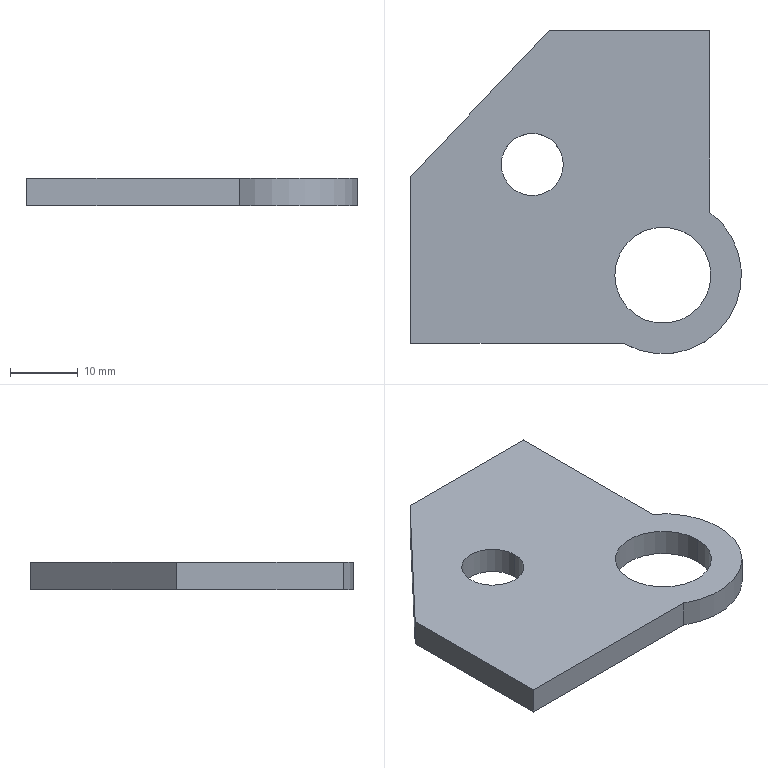Component | SolidWorks | MirrorRearSidePlate1-2 | 1 solid | 12 faces | box 48.87 x 47.78 x 4 mm | volume 6683 mm3 | plane 7 | cylinder 5 | commonest cylinder face diameters 9.176 x2 14.2 x2 23.231 x1
STEP:
#1=CARTESIAN_POINT('',(7.015,0.1706,-0.9252));
#2=VERTEX_POINT('',#1);
#3=CARTESIAN_POINT('',(6.653,0.1706,-0.9252));
#4=VERTEX_POINT('',#3);
#5=CARTESIAN_POINT('',(6.834,0.1706,-0.9252));
#6=DIRECTION('',(0.,0.,1.));
#7=DIRECTION('',(1.,0.,0.));
#8=AXIS2_PLACEMENT_3D('',#5,#6,#7);
#9=CIRCLE('',#8,0.1806);
#10=EDGE_CURVE('',#2,#4,#9,.T.);
#11=ORIENTED_EDGE('',*,*,#10,.F.);
#12=CARTESIAN_POINT('',(7.015,0.1706,-0.7677));
#13=VERTEX_POINT('',#12);
#14=CARTESIAN_POINT('',(7.015,0.1706,-0.9252));
#15=DIRECTION('',(0.,0.,1.));
#16=VECTOR('',#15,39.37);
#17=LINE('',#14,#16);
#18=EDGE_CURVE('',#2,#13,#17,.T.);
#19=ORIENTED_EDGE('',*,*,#18,.T.);
#20=CARTESIAN_POINT('',(6.653,0.1706,-0.7677));
#21=VERTEX_POINT('',#20);
#22=CARTESIAN_POINT('',(6.834,0.1706,-0.7677));
#23=DIRECTION('',(0.,0.,1.));
#24=DIRECTION('',(1.,0.,0.));
#25=AXIS2_PLACEMENT_3D('',#22,#23,#24);
#26=CIRCLE('',#25,0.1806);
#27=EDGE_CURVE('',#13,#21,#26,.T.);
#28=ORIENTED_EDGE('',*,*,#27,.T.);
#29=CARTESIAN_POINT('',(6.653,0.1706,-0.9252));
#30=DIRECTION('',(0.,0.,1.));
#31=VECTOR('',#30,39.37);
#32=LINE('',#29,#31);
#33=EDGE_CURVE('',#4,#21,#32,.T.);
#34=ORIENTED_EDGE('',*,*,#33,.F.);
#35=EDGE_LOOP('',(#11,#19,#28,#34));
#36=FACE_OUTER_BOUND('',#35,.T.);
#37=CARTESIAN_POINT('',(6.834,0.1706,-0.9252));
#38=DIRECTION('',(0.,0.,1.));
#39=DIRECTION('',(-1.,0.,0.));
#40=AXIS2_PLACEMENT_3D('',#37,#38,#39);
#41=CYLINDRICAL_SURFACE('',#40,0.1806);
#42=ADVANCED_FACE('',(#36),#41,.F.);
#43=CARTESIAN_POINT('',(7.873,-0.4733,-0.9252));
#44=VERTEX_POINT('',#43);
#45=CARTESIAN_POINT('',(7.314,-0.4733,-0.9252));
#46=VERTEX_POINT('',#45);
#47=CARTESIAN_POINT('',(7.594,-0.4733,-0.9252));
#48=DIRECTION('',(0.,0.,1.));
#49=DIRECTION('',(1.,0.,0.));
#50=AXIS2_PLACEMENT_3D('',#47,#48,#49);
#51=CIRCLE('',#50,0.2795);
#52=EDGE_CURVE('',#44,#46,#51,.T.);
#53=ORIENTED_EDGE('',*,*,#52,.F.);
#54=CARTESIAN_POINT('',(7.873,-0.4733,-0.7677));
#55=VERTEX_POINT('',#54);
#56=CARTESIAN_POINT('',(7.873,-0.4733,-0.9252));
#57=DIRECTION('',(0.,0.,1.));
#58=VECTOR('',#57,39.37);
#59=LINE('',#56,#58);
#60=EDGE_CURVE('',#44,#55,#59,.T.);
#61=ORIENTED_EDGE('',*,*,#60,.T.);
#62=CARTESIAN_POINT('',(7.314,-0.4733,-0.7677));
#63=VERTEX_POINT('',#62);
#64=CARTESIAN_POINT('',(7.594,-0.4733,-0.7677));
#65=DIRECTION('',(0.,0.,1.));
#66=DIRECTION('',(1.,0.,0.));
#67=AXIS2_PLACEMENT_3D('',#64,#65,#66);
#68=CIRCLE('',#67,0.2795);
#69=EDGE_CURVE('',#55,#63,#68,.T.);
#70=ORIENTED_EDGE('',*,*,#69,.T.);
#71=CARTESIAN_POINT('',(7.314,-0.4733,-0.9252));
#72=DIRECTION('',(0.,0.,1.));
#73=VECTOR('',#72,39.37);
#74=LINE('',#71,#73);
#75=EDGE_CURVE('',#46,#63,#74,.T.);
#76=ORIENTED_EDGE('',*,*,#75,.F.);
#77=EDGE_LOOP('',(#53,#61,#70,#76));
#78=FACE_OUTER_BOUND('',#77,.T.);
#79=CARTESIAN_POINT('',(7.594,-0.4733,-0.9252));
#80=DIRECTION('',(0.,0.,1.));
#81=DIRECTION('',(-1.,0.,0.));
#82=AXIS2_PLACEMENT_3D('',#79,#80,#81);
#83=CYLINDRICAL_SURFACE('',#82,0.2795);
#84=ADVANCED_FACE('',(#78),#83,.F.);
#85=CARTESIAN_POINT('',(6.933,0.9504,-0.9252));
#86=VERTEX_POINT('',#85);
#87=CARTESIAN_POINT('',(6.127,0.1014,-0.9252));
#88=VERTEX_POINT('',#87);
#89=CARTESIAN_POINT('',(6.127,0.1014,-0.9252));
#90=DIRECTION('',(-0.6886,-0.7251,0.));
#91=VECTOR('',#90,39.37);
#92=LINE('',#89,#91);
#93=EDGE_CURVE('',#86,#88,#92,.T.);
#94=ORIENTED_EDGE('',*,*,#93,.F.);
#95=CARTESIAN_POINT('',(7.867,0.9504,-0.9252));
#96=VERTEX_POINT('',#95);
#97=CARTESIAN_POINT('',(6.933,0.9504,-0.9252));
#98=DIRECTION('',(-1.,0.,0.));
#99=VECTOR('',#98,39.37);
#100=LINE('',#97,#99);
#101=EDGE_CURVE('',#96,#86,#100,.T.);
#102=ORIENTED_EDGE('',*,*,#101,.F.);
#103=CARTESIAN_POINT('',(7.867,-0.107,-0.9252));
#104=VERTEX_POINT('',#103);
#105=CARTESIAN_POINT('',(7.867,0.9504,-0.9252));
#106=DIRECTION('',(0.,1.,0.));
#107=VECTOR('',#106,39.37);
#108=LINE('',#105,#107);
#109=EDGE_CURVE('',#104,#96,#108,.T.);
#110=ORIENTED_EDGE('',*,*,#109,.F.);
#111=CARTESIAN_POINT('',(7.365,-0.8697,-0.9252));
#112=VERTEX_POINT('',#111);
#113=CARTESIAN_POINT('',(7.594,-0.4733,-0.9252));
#114=DIRECTION('',(0.,0.,1.));
#115=DIRECTION('',(-1.,0.,0.));
#116=AXIS2_PLACEMENT_3D('',#113,#114,#115);
#117=CIRCLE('',#116,0.4573);
#118=EDGE_CURVE('',#112,#104,#117,.T.);
#119=ORIENTED_EDGE('',*,*,#118,.F.);
#120=CARTESIAN_POINT('',(6.127,-0.8697,-0.9252));
#121=VERTEX_POINT('',#120);
#122=CARTESIAN_POINT('',(6.127,-0.8697,-0.9252));
#123=DIRECTION('',(1.,0.,0.));
#124=VECTOR('',#123,39.37);
#125=LINE('',#122,#124);
#126=EDGE_CURVE('',#121,#112,#125,.T.);
#127=ORIENTED_EDGE('',*,*,#126,.F.);
#128=CARTESIAN_POINT('',(6.127,0.1014,-0.9252));
#129=DIRECTION('',(0.,-1.,0.));
#130=VECTOR('',#129,39.37);
#131=LINE('',#128,#130);
#132=EDGE_CURVE('',#88,#121,#131,.T.);
#133=ORIENTED_EDGE('',*,*,#132,.F.);
#134=EDGE_LOOP('',(#94,#102,#110,#119,#127,#133));
#135=FACE_OUTER_BOUND('',#134,.T.);
#136=CARTESIAN_POINT('',(7.594,-0.4733,-0.9252));
#137=DIRECTION('',(0.,0.,1.));
#138=DIRECTION('',(1.,0.,0.));
#139=AXIS2_PLACEMENT_3D('',#136,#137,#138);
#140=CIRCLE('',#139,0.2795);
#141=EDGE_CURVE('',#46,#44,#140,.T.);
#142=ORIENTED_EDGE('',*,*,#141,.T.);
#143=ORIENTED_EDGE('',*,*,#52,.T.);
#144=EDGE_LOOP('',(#142,#143));
#145=FACE_BOUND('',#144,.T.);
#146=CARTESIAN_POINT('',(6.834,0.1706,-0.9252));
#147=DIRECTION('',(0.,0.,1.));
#148=DIRECTION('',(1.,0.,0.));
#149=AXIS2_PLACEMENT_3D('',#146,#147,#148);
#150=CIRCLE('',#149,0.1806);
#151=EDGE_CURVE('',#4,#2,#150,.T.);
#152=ORIENTED_EDGE('',*,*,#151,.T.);
#153=ORIENTED_EDGE('',*,*,#10,.T.);
#154=EDGE_LOOP('',(#152,#153));
#155=FACE_BOUND('',#154,.T.);
#156=CARTESIAN_POINT('',(7.594,-0.4733,-0.9252));
#157=DIRECTION('',(0.,0.,1.));
#158=DIRECTION('',(-1.,0.,0.));
#159=AXIS2_PLACEMENT_3D('',#156,#157,#158);
#160=PLANE('',#159);
#161=ADVANCED_FACE('',(#135,#145,#155),#160,.F.);
#162=CARTESIAN_POINT('',(7.594,-0.4733,-0.7677));
#163=DIRECTION('',(0.,0.,1.));
#164=DIRECTION('',(1.,0.,0.));
#165=AXIS2_PLACEMENT_3D('',#162,#163,#164);
#166=CIRCLE('',#165,0.2795);
#167=EDGE_CURVE('',#63,#55,#166,.T.);
#168=ORIENTED_EDGE('',*,*,#167,.F.);
#169=ORIENTED_EDGE('',*,*,#69,.F.);
#170=EDGE_LOOP('',(#168,#169));
#171=FACE_BOUND('',#170,.T.);
#172=CARTESIAN_POINT('',(6.933,0.9504,-0.7677));
#173=VERTEX_POINT('',#172);
#174=CARTESIAN_POINT('',(6.127,0.1014,-0.7677));
#175=VERTEX_POINT('',#174);
#176=CARTESIAN_POINT('',(6.127,0.1014,-0.7677));
#177=DIRECTION('',(-0.6886,-0.7251,0.));
#178=VECTOR('',#177,39.37);
#179=LINE('',#176,#178);
#180=EDGE_CURVE('',#173,#175,#179,.T.);
#181=ORIENTED_EDGE('',*,*,#180,.T.);
#182=CARTESIAN_POINT('',(6.127,-0.8697,-0.7677));
#183=VERTEX_POINT('',#182);
#184=CARTESIAN_POINT('',(6.127,0.1014,-0.7677));
#185=DIRECTION('',(0.,-1.,0.));
#186=VECTOR('',#185,39.37);
#187=LINE('',#184,#186);
#188=EDGE_CURVE('',#175,#183,#187,.T.);
#189=ORIENTED_EDGE('',*,*,#188,.T.);
#190=CARTESIAN_POINT('',(7.365,-0.8697,-0.7677));
#191=VERTEX_POINT('',#190);
#192=CARTESIAN_POINT('',(6.127,-0.8697,-0.7677));
#193=DIRECTION('',(1.,0.,0.));
#194=VECTOR('',#193,39.37);
#195=LINE('',#192,#194);
#196=EDGE_CURVE('',#183,#191,#195,.T.);
#197=ORIENTED_EDGE('',*,*,#196,.T.);
#198=CARTESIAN_POINT('',(7.867,-0.107,-0.7677));
#199=VERTEX_POINT('',#198);
#200=CARTESIAN_POINT('',(7.594,-0.4733,-0.7677));
#201=DIRECTION('',(0.,0.,1.));
#202=DIRECTION('',(-1.,0.,0.));
#203=AXIS2_PLACEMENT_3D('',#200,#201,#202);
#204=CIRCLE('',#203,0.4573);
#205=EDGE_CURVE('',#191,#199,#204,.T.);
#206=ORIENTED_EDGE('',*,*,#205,.T.);
#207=CARTESIAN_POINT('',(7.867,0.9504,-0.7677));
#208=VERTEX_POINT('',#207);
#209=CARTESIAN_POINT('',(7.867,0.9504,-0.7677));
#210=DIRECTION('',(0.,1.,0.));
#211=VECTOR('',#210,39.37);
#212=LINE('',#209,#211);
#213=EDGE_CURVE('',#199,#208,#212,.T.);
#214=ORIENTED_EDGE('',*,*,#213,.T.);
#215=CARTESIAN_POINT('',(6.933,0.9504,-0.7677));
#216=DIRECTION('',(-1.,0.,0.));
#217=VECTOR('',#216,39.37);
#218=LINE('',#215,#217);
#219=EDGE_CURVE('',#208,#173,#218,.T.);
#220=ORIENTED_EDGE('',*,*,#219,.T.);
#221=EDGE_LOOP('',(#181,#189,#197,#206,#214,#220));
#222=FACE_OUTER_BOUND('',#221,.T.);
#223=CARTESIAN_POINT('',(6.834,0.1706,-0.7677));
#224=DIRECTION('',(0.,0.,1.));
#225=DIRECTION('',(1.,0.,0.));
#226=AXIS2_PLACEMENT_3D('',#223,#224,#225);
#227=CIRCLE('',#226,0.1806);
#228=EDGE_CURVE('',#21,#13,#227,.T.);
#229=ORIENTED_EDGE('',*,*,#228,.F.);
#230=ORIENTED_EDGE('',*,*,#27,.F.);
#231=EDGE_LOOP('',(#229,#230));
#232=FACE_BOUND('',#231,.T.);
#233=CARTESIAN_POINT('',(7.594,-0.4733,-0.7677));
#234=DIRECTION('',(0.,0.,1.));
#235=DIRECTION('',(-1.,0.,0.));
#236=AXIS2_PLACEMENT_3D('',#233,#234,#235);
#237=PLANE('',#236);
#238=ADVANCED_FACE('',(#171,#222,#232),#237,.T.);
#239=ORIENTED_EDGE('',*,*,#180,.F.);
#240=CARTESIAN_POINT('',(6.933,0.9504,-0.9252));
#241=DIRECTION('',(0.,0.,1.));
#242=VECTOR('',#241,39.37);
#243=LINE('',#240,#242);
#244=EDGE_CURVE('',#86,#173,#243,.T.);
#245=ORIENTED_EDGE('',*,*,#244,.F.);
#246=ORIENTED_EDGE('',*,*,#93,.T.);
#247=CARTESIAN_POINT('',(6.127,0.1014,-0.9252));
#248=DIRECTION('',(0.,0.,1.));
#249=VECTOR('',#248,39.37);
#250=LINE('',#247,#249);
#251=EDGE_CURVE('',#88,#175,#250,.T.);
#252=ORIENTED_EDGE('',*,*,#251,.T.);
#253=EDGE_LOOP('',(#239,#245,#246,#252));
#254=FACE_OUTER_BOUND('',#253,.T.);
#255=CARTESIAN_POINT('',(6.127,0.1014,-0.9252));
#256=DIRECTION('',(0.7251,-0.6886,0.));
#257=DIRECTION('',(0.6886,0.7251,0.));
#258=AXIS2_PLACEMENT_3D('',#255,#256,#257);
#259=PLANE('',#258);
#260=ADVANCED_FACE('',(#254),#259,.F.);
#261=ORIENTED_EDGE('',*,*,#188,.F.);
#262=ORIENTED_EDGE('',*,*,#251,.F.);
#263=ORIENTED_EDGE('',*,*,#132,.T.);
#264=CARTESIAN_POINT('',(6.127,-0.8697,-0.9252));
#265=DIRECTION('',(0.,0.,1.));
#266=VECTOR('',#265,39.37);
#267=LINE('',#264,#266);
#268=EDGE_CURVE('',#121,#183,#267,.T.);
#269=ORIENTED_EDGE('',*,*,#268,.T.);
#270=EDGE_LOOP('',(#261,#262,#263,#269));
#271=FACE_OUTER_BOUND('',#270,.T.);
#272=CARTESIAN_POINT('',(6.127,0.1014,-0.9252));
#273=DIRECTION('',(1.,0.,0.));
#274=DIRECTION('',(0.,0.,1.));
#275=AXIS2_PLACEMENT_3D('',#272,#273,#274);
#276=PLANE('',#275);
#277=ADVANCED_FACE('',(#271),#276,.F.);
#278=ORIENTED_EDGE('',*,*,#196,.F.);
#279=ORIENTED_EDGE('',*,*,#268,.F.);
#280=ORIENTED_EDGE('',*,*,#126,.T.);
#281=CARTESIAN_POINT('',(7.365,-0.8697,-0.9252));
#282=DIRECTION('',(0.,0.,1.));
#283=VECTOR('',#282,39.37);
#284=LINE('',#281,#283);
#285=EDGE_CURVE('',#112,#191,#284,.T.);
#286=ORIENTED_EDGE('',*,*,#285,.T.);
#287=EDGE_LOOP('',(#278,#279,#280,#286));
#288=FACE_OUTER_BOUND('',#287,.T.);
#289=CARTESIAN_POINT('',(6.127,-0.8697,-0.9252));
#290=DIRECTION('',(0.,1.,0.));
#291=DIRECTION('',(0.,0.,-1.));
#292=AXIS2_PLACEMENT_3D('',#289,#290,#291);
#293=PLANE('',#292);
#294=ADVANCED_FACE('',(#288),#293,.F.);
#295=ORIENTED_EDGE('',*,*,#205,.F.);
#296=ORIENTED_EDGE('',*,*,#285,.F.);
#297=ORIENTED_EDGE('',*,*,#118,.T.);
#298=CARTESIAN_POINT('',(7.867,-0.107,-0.9252));
#299=DIRECTION('',(0.,0.,1.));
#300=VECTOR('',#299,39.37);
#301=LINE('',#298,#300);
#302=EDGE_CURVE('',#104,#199,#301,.T.);
#303=ORIENTED_EDGE('',*,*,#302,.T.);
#304=EDGE_LOOP('',(#295,#296,#297,#303));
#305=FACE_OUTER_BOUND('',#304,.T.);
#306=CARTESIAN_POINT('',(7.594,-0.4733,-0.9252));
#307=DIRECTION('',(0.,0.,1.));
#308=DIRECTION('',(-1.,0.,0.));
#309=AXIS2_PLACEMENT_3D('',#306,#307,#308);
#310=CYLINDRICAL_SURFACE('',#309,0.4573);
#311=ADVANCED_FACE('',(#305),#310,.T.);
#312=ORIENTED_EDGE('',*,*,#213,.F.);
#313=ORIENTED_EDGE('',*,*,#302,.F.);
#314=ORIENTED_EDGE('',*,*,#109,.T.);
#315=CARTESIAN_POINT('',(7.867,0.9504,-0.9252));
#316=DIRECTION('',(0.,0.,1.));
#317=VECTOR('',#316,39.37);
#318=LINE('',#315,#317);
#319=EDGE_CURVE('',#96,#208,#318,.T.);
#320=ORIENTED_EDGE('',*,*,#319,.T.);
#321=EDGE_LOOP('',(#312,#313,#314,#320));
#322=FACE_OUTER_BOUND('',#321,.T.);
#323=CARTESIAN_POINT('',(7.867,0.9504,-0.9252));
#324=DIRECTION('',(-1.,0.,0.));
#325=DIRECTION('',(0.,0.,-1.));
#326=AXIS2_PLACEMENT_3D('',#323,#324,#325);
#327=PLANE('',#326);
#328=ADVANCED_FACE('',(#322),#327,.F.);
#329=ORIENTED_EDGE('',*,*,#219,.F.);
#330=ORIENTED_EDGE('',*,*,#319,.F.);
#331=ORIENTED_EDGE('',*,*,#101,.T.);
#332=ORIENTED_EDGE('',*,*,#244,.T.);
#333=EDGE_LOOP('',(#329,#330,#331,#332));
#334=FACE_OUTER_BOUND('',#333,.T.);
#335=CARTESIAN_POINT('',(6.933,0.9504,-0.9252));
#336=DIRECTION('',(0.,-1.,0.));
#337=DIRECTION('',(0.,0.,1.));
#338=AXIS2_PLACEMENT_3D('',#335,#336,#337);
#339=PLANE('',#338);
#340=ADVANCED_FACE('',(#334),#339,.F.);
#341=ORIENTED_EDGE('',*,*,#60,.F.);
#342=ORIENTED_EDGE('',*,*,#141,.F.);
#343=ORIENTED_EDGE('',*,*,#75,.T.);
#344=ORIENTED_EDGE('',*,*,#167,.T.);
#345=EDGE_LOOP('',(#341,#342,#343,#344));
#346=FACE_OUTER_BOUND('',#345,.T.);
#347=CARTESIAN_POINT('',(7.594,-0.4733,-0.9252));
#348=DIRECTION('',(0.,0.,1.));
#349=DIRECTION('',(-1.,0.,0.));
#350=AXIS2_PLACEMENT_3D('',#347,#348,#349);
#351=CYLINDRICAL_SURFACE('',#350,0.2795);
#352=ADVANCED_FACE('',(#346),#351,.F.);
#353=ORIENTED_EDGE('',*,*,#18,.F.);
#354=ORIENTED_EDGE('',*,*,#151,.F.);
#355=ORIENTED_EDGE('',*,*,#33,.T.);
#356=ORIENTED_EDGE('',*,*,#228,.T.);
#357=EDGE_LOOP('',(#353,#354,#355,#356));
#358=FACE_OUTER_BOUND('',#357,.T.);
#359=CARTESIAN_POINT('',(6.834,0.1706,-0.9252));
#360=DIRECTION('',(0.,0.,1.));
#361=DIRECTION('',(-1.,0.,0.));
#362=AXIS2_PLACEMENT_3D('',#359,#360,#361);
#363=CYLINDRICAL_SURFACE('',#362,0.1806);
#364=ADVANCED_FACE('',(#358),#363,.F.);
#365=CLOSED_SHELL('',(#42,#84,#161,#238,#260,#277,#294,#311,#328,#340,#352,#364));
#366=MANIFOLD_SOLID_BREP('',#365);
#367=CARTESIAN_POINT('',(0.,0.,0.));
#368=DIRECTION('',(0.,0.,1.));
#369=DIRECTION('',(1.,0.,0.));
#370=AXIS2_PLACEMENT_3D('',#367,#368,#369);
#371=(LENGTH_UNIT()NAMED_UNIT(*)SI_UNIT($,.METRE.));
#372=LENGTH_MEASURE_WITH_UNIT(LENGTH_MEASURE(0.0254),#371);
#373=DIMENSIONAL_EXPONENTS(1.,0.,0.,0.,0.,0.,0.);
#374=(CONVERSION_BASED_UNIT('',#372)LENGTH_UNIT()NAMED_UNIT(#373));
#375=UNCERTAINTY_MEASURE_WITH_UNIT(LENGTH_MEASURE(0.00001),#374,'','');
#376=(NAMED_UNIT(*)PLANE_ANGLE_UNIT()SI_UNIT($,.RADIAN.));
#377=(NAMED_UNIT(*)SI_UNIT($,.STERADIAN.)SOLID_ANGLE_UNIT());
#378=(GEOMETRIC_REPRESENTATION_CONTEXT(3)GLOBAL_UNCERTAINTY_ASSIGNED_CONTEXT((#375))GLOBAL_UNIT_ASSIGNED_CONTEXT((#374,#376,#377))REPRESENTATION_CONTEXT('',''));
#379=ADVANCED_BREP_SHAPE_REPRESENTATION('',(#366,#370),#378);
#380=COLOUR_RGB('',0.7922,0.8196,0.9333);
#381=FILL_AREA_STYLE_COLOUR('',#380);
#382=FILL_AREA_STYLE('',(#381));
#383=SURFACE_STYLE_FILL_AREA(#382);
#384=SURFACE_SIDE_STYLE('',(#383));
#385=SURFACE_STYLE_USAGE(.BOTH.,#384);
#386=PRESENTATION_STYLE_ASSIGNMENT((#385));
#387=STYLED_ITEM('',(#386),#366);
#388=PRESENTATION_LAYER_ASSIGNMENT('','',(#387));
#389=(LENGTH_UNIT()NAMED_UNIT(*)SI_UNIT($,.METRE.));
#390=LENGTH_MEASURE_WITH_UNIT(LENGTH_MEASURE(0.0254),#389);
#391=DIMENSIONAL_EXPONENTS(1.,0.,0.,0.,0.,0.,0.);
#392=(CONVERSION_BASED_UNIT('',#390)LENGTH_UNIT()NAMED_UNIT(#391));
#393=UNCERTAINTY_MEASURE_WITH_UNIT(LENGTH_MEASURE(0.00001),#392,'','');
#394=(NAMED_UNIT(*)PLANE_ANGLE_UNIT()SI_UNIT($,.RADIAN.));
#395=(NAMED_UNIT(*)SI_UNIT($,.STERADIAN.)SOLID_ANGLE_UNIT());
#396=(GEOMETRIC_REPRESENTATION_CONTEXT(3)GLOBAL_UNCERTAINTY_ASSIGNED_CONTEXT((#393))GLOBAL_UNIT_ASSIGNED_CONTEXT((#392,#394,#395))REPRESENTATION_CONTEXT('',''));
#397=MECHANICAL_DESIGN_GEOMETRIC_PRESENTATION_REPRESENTATION('',(#387),#396);